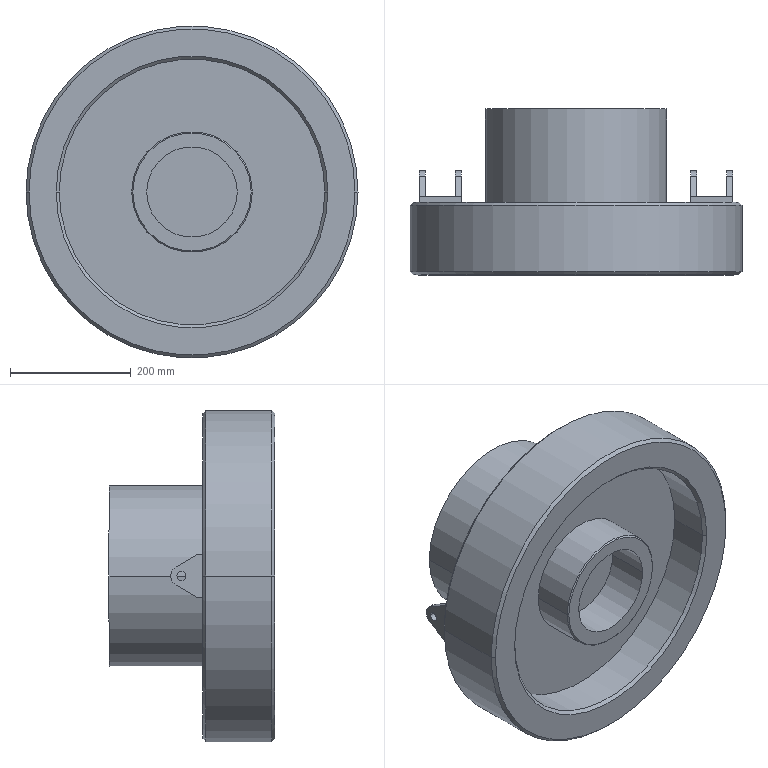Component | SolidWorks | Z-AxisBase-2 | 2 solids | 67 faces | box 550 x 275 x 550 mm | volume 25944172 mm3 | plane 31 | cylinder 28 | cone 8 | commonest cylinder face diameters 15 x8 35 x6 200 x2 150 x2 440 x2 550 x2 190 x2 300 x2
build123d program:
from build123d import *

# Parameters (mm, degrees)
SKETCH1_R                = 35
BOSS_EXTRUDE1_DEPTH      = 80
BOSS_EXTRUDE2_DEPTH      = 70
BOSS_EXTRUDE2_DEPTH_BACK = 80
SKETCH2_R                = 150
SKETCH2_R_2              = 95
SKETCH3_R                = 150
BOSS_EXTRUDE3_DEPTH      = 5
SKETCH4_R                = 275
BOSS_EXTRUDE4_DEPTH      = 50
SKETCH5_R                = 275
SKETCH5_R_2              = 220
SKETCH5_R_3              = 100
SKETCH5_R_4              = 75
BOSS_EXTRUDE5_DEPTH      = 70
SKETCH7_W                = 70
SKETCH7_H                = 70
BOSS_EXTRUDE6_DEPTH      = 10
SKETCH8_4_R              = 7.5
BOSS_EXTRUDE7_DEPTH      = 10
BOSS_EXTRUDE8_START      = -70
SKETCH8_2_R              = 7.5
BOSS_EXTRUDE8_DEPTH      = 10
BOSS_EXTRUDE9_START      = -520
SKETCH8_3_R              = 7.5
BOSS_EXTRUDE9_DEPTH      = 10
BOSS_EXTRUDE10_START     = -450
SKETCH8_4_2_R            = 7.5
BOSS_EXTRUDE10_DEPTH     = 10
CHAMFER1_SIZE            = 2
CHAMFER2_SIZE            = 5


with BuildPart() as part:
    # Sketch1 → Boss-Extrude1 (new body)
    with BuildSketch(Plane.XY):
        with Locations((0, 300)):
            Circle(SKETCH1_R)
    extrude(amount=BOSS_EXTRUDE1_DEPTH)


with BuildPart() as body_2:
    # Sketch2 → Boss-Extrude2 (new, two sides: drawn at the far end of the back side and taken through both)
    with BuildSketch(Plane.XY.offset(80).offset(-BOSS_EXTRUDE2_DEPTH_BACK)):
        with Locations((0, 300)):
            Circle(SKETCH2_R)
        with Locations((0, 300)):
            Circle(SKETCH2_R_2, mode=Mode.SUBTRACT)
    extrude(amount=BOSS_EXTRUDE2_DEPTH + BOSS_EXTRUDE2_DEPTH_BACK)

    # Sketch3 → Boss-Extrude3 (add)
    with BuildSketch(Plane.XY.offset(150)):
        with Locations((0, 300)):
            Circle(SKETCH3_R)
    extrude(amount=BOSS_EXTRUDE3_DEPTH)

    # Sketch4 → Boss-Extrude4 (add)
    with BuildSketch(Plane.XY.offset(155)):
        with Locations((0, 300)):
            Circle(SKETCH4_R)
    extrude(amount=BOSS_EXTRUDE4_DEPTH)

    # Sketch5 → Boss-Extrude5 (add)
    # profile 1 of 2: a face of its own
    with BuildSketch(Plane.XY.offset(205)):
        with Locations((0, 300)):
            Circle(SKETCH5_R)
        with Locations((0, 300)):
            Circle(SKETCH5_R_2, mode=Mode.SUBTRACT)
    # profile 2 of 2: a face of its own
    with BuildSketch(Plane.XY.offset(205)):
        with Locations((0, 300)):
            Circle(SKETCH5_R_3)
        with Locations((0, 300)):
            Circle(SKETCH5_R_4, mode=Mode.SUBTRACT)
    extrude(amount=BOSS_EXTRUDE5_DEPTH)

    # Sketch7 → Boss-Extrude6 (add)
    with BuildSketch(Plane(origin=(0, 0, 155), x_dir=(-1, 0, 0), z_dir=(0, 0, -1))):
        with Locations((225, 300)):
            Rectangle(SKETCH7_W, SKETCH7_H)
        with Locations((-225, 300)):
            Rectangle(SKETCH7_W, SKETCH7_H)
    extrude(amount=BOSS_EXTRUDE6_DEPTH)

    # Sketch8_4 → Boss-Extrude7 (add)
    with BuildSketch(Plane(origin=(260, 0, 0), x_dir=(0, 0, -1), z_dir=(1, 0, 0))):
        with BuildLine():
            Line((-145, 335), (-111.13, 315.086))
            ThreePointArc((-111.13, 315.086), (-102.5, 300), (-111.13, 284.914))
            Line((-111.13, 284.914), (-145, 265))
            Line((-145, 265), (-145, 335))
        make_face()
        with Locations((-120, 300)):
            Circle(SKETCH8_4_R, mode=Mode.SUBTRACT)
    extrude(amount=-BOSS_EXTRUDE7_DEPTH)

    # Sketch8_2 → Boss-Extrude8 (add)
    with BuildSketch(Plane(origin=(260, 0, 0), x_dir=(0, 0, -1), z_dir=(1, 0, 0)).offset(BOSS_EXTRUDE8_START)):
        with BuildLine():
            Line((-145, 335), (-111.13, 315.086))
            ThreePointArc((-111.13, 315.086), (-102.5, 300), (-111.13, 284.914))
            Line((-111.13, 284.914), (-145, 265))
            Line((-145, 265), (-145, 335))
        make_face()
        with Locations((-120, 300)):
            Circle(SKETCH8_2_R, mode=Mode.SUBTRACT)
    extrude(amount=BOSS_EXTRUDE8_DEPTH)

    # Sketch8_3 → Boss-Extrude9 (add)
    with BuildSketch(Plane(origin=(260, 0, 0), x_dir=(0, 0, -1), z_dir=(1, 0, 0)).offset(BOSS_EXTRUDE9_START)):
        with BuildLine():
            Line((-145, 335), (-111.13, 315.086))
            ThreePointArc((-111.13, 315.086), (-102.5, 300), (-111.13, 284.914))
            Line((-111.13, 284.914), (-145, 265))
            Line((-145, 265), (-145, 335))
        make_face()
        with Locations((-120, 300)):
            Circle(SKETCH8_3_R, mode=Mode.SUBTRACT)
    extrude(amount=BOSS_EXTRUDE9_DEPTH)

    # Sketch8_4 2 → Boss-Extrude10 (add)
    with BuildSketch(Plane(origin=(260, 0, 0), x_dir=(0, 0, -1), z_dir=(1, 0, 0)).offset(BOSS_EXTRUDE10_START)):
        with BuildLine():
            Line((-145, 335), (-111.13, 315.086))
            ThreePointArc((-111.13, 315.086), (-102.5, 300), (-111.13, 284.914))
            Line((-111.13, 284.914), (-145, 265))
            Line((-145, 265), (-145, 335))
        make_face()
        with Locations((-120, 300)):
            Circle(SKETCH8_4_2_R, mode=Mode.SUBTRACT)
    extrude(amount=-BOSS_EXTRUDE10_DEPTH)

    # Chamfer1
    chamfer1_edges = [body_2.edges().sort_by_distance(p)[0] for p in [
        (-100, 300, 275),
    ]]
    chamfer(chamfer1_edges, length=CHAMFER1_SIZE)

    # Chamfer2
    chamfer2_edges = [body_2.edges().sort_by_distance(p)[0] for p in [
        (-275, 300, 155),
        (-220, 300, 275),
        (-275, 300, 275),
    ]]
    chamfer(chamfer2_edges, length=CHAMFER2_SIZE)


solid = Compound([part.part, body_2.part])

# Placed as in the assembly
solid = solid.moved(Location((0, -256, -600), (90, 0, 0)))